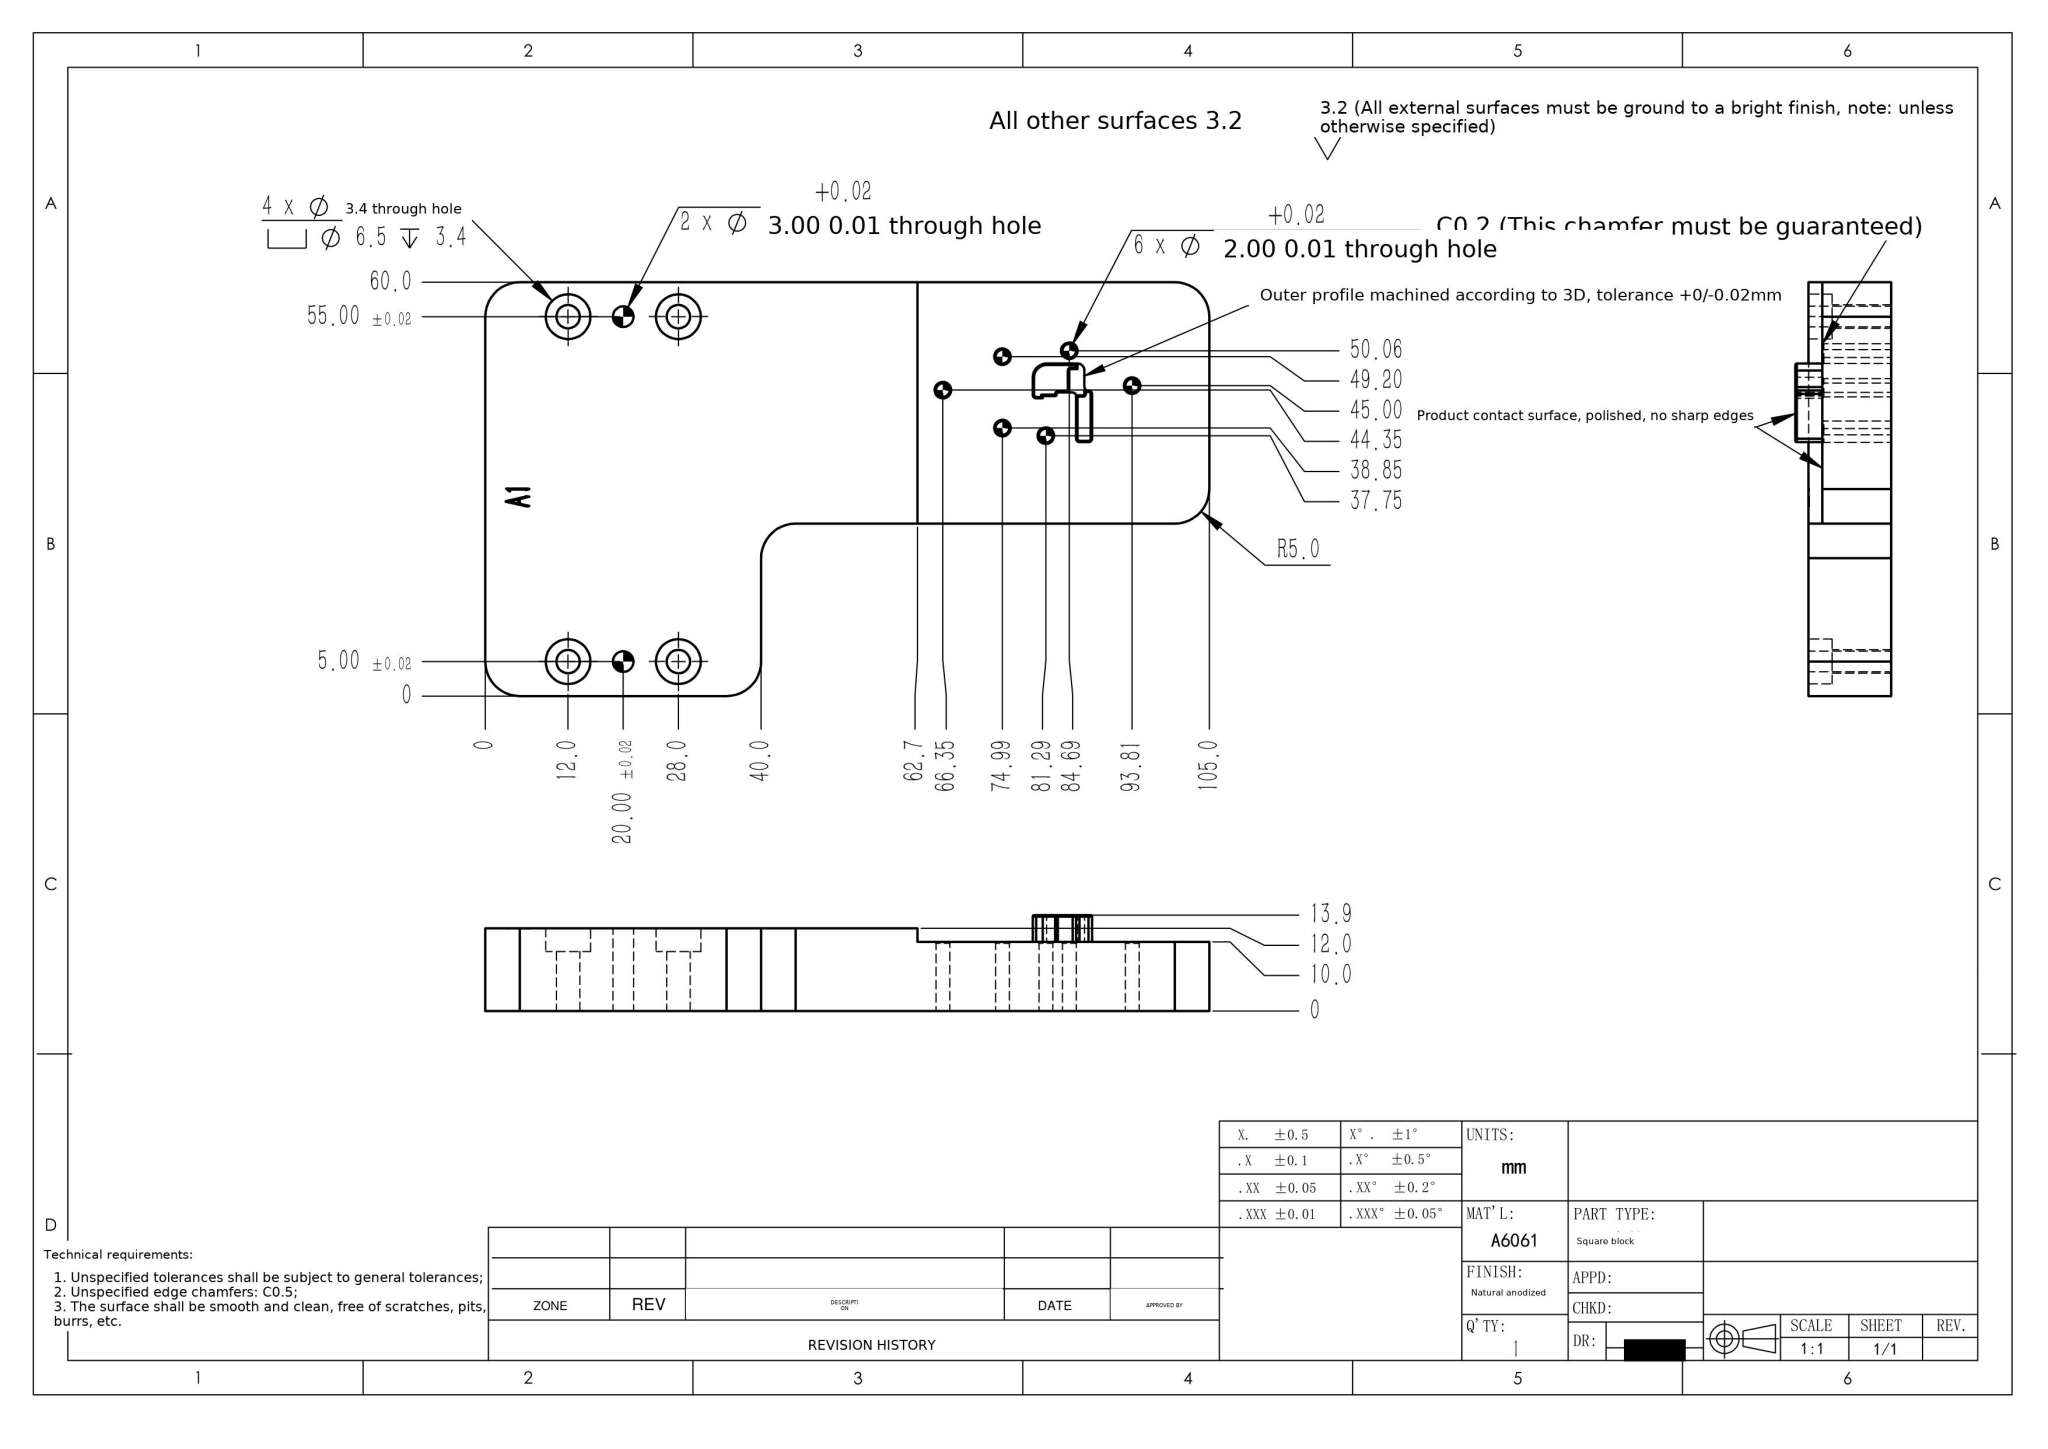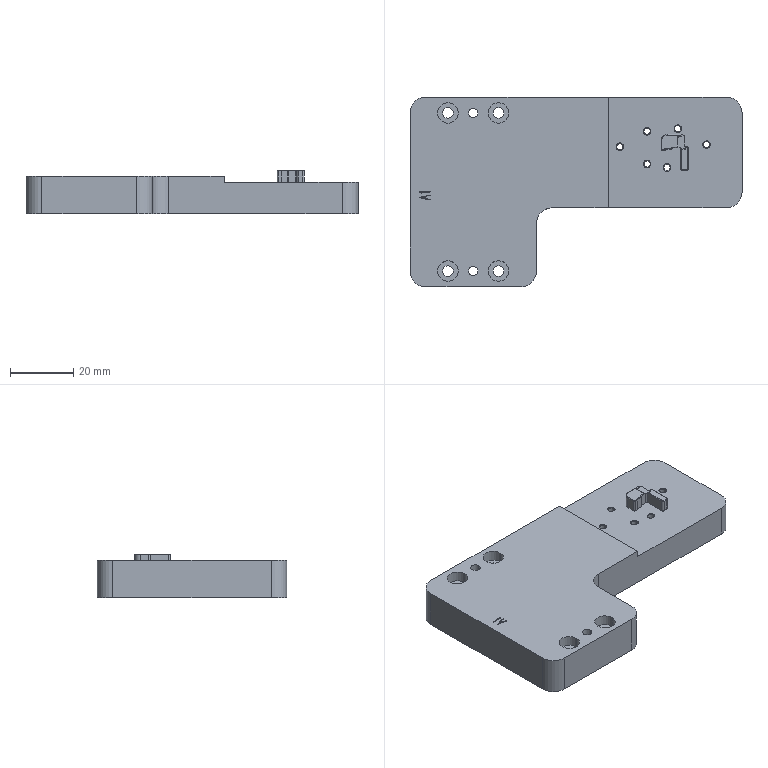Part | SolidWorks | mm | material A6061 | 1 solid | 156 faces | box 105 x 60 x 13.9 mm | volume 51971 mm3 | cylinder 64 | plane 59 | cone 12 | spline 11 | torus 9 | sphere 1 | commonest cylinder face diameters 0.4 x18 2 x13 6.5 x8 3.4 x8 1 x6 10 x6 3 x4 4 x1